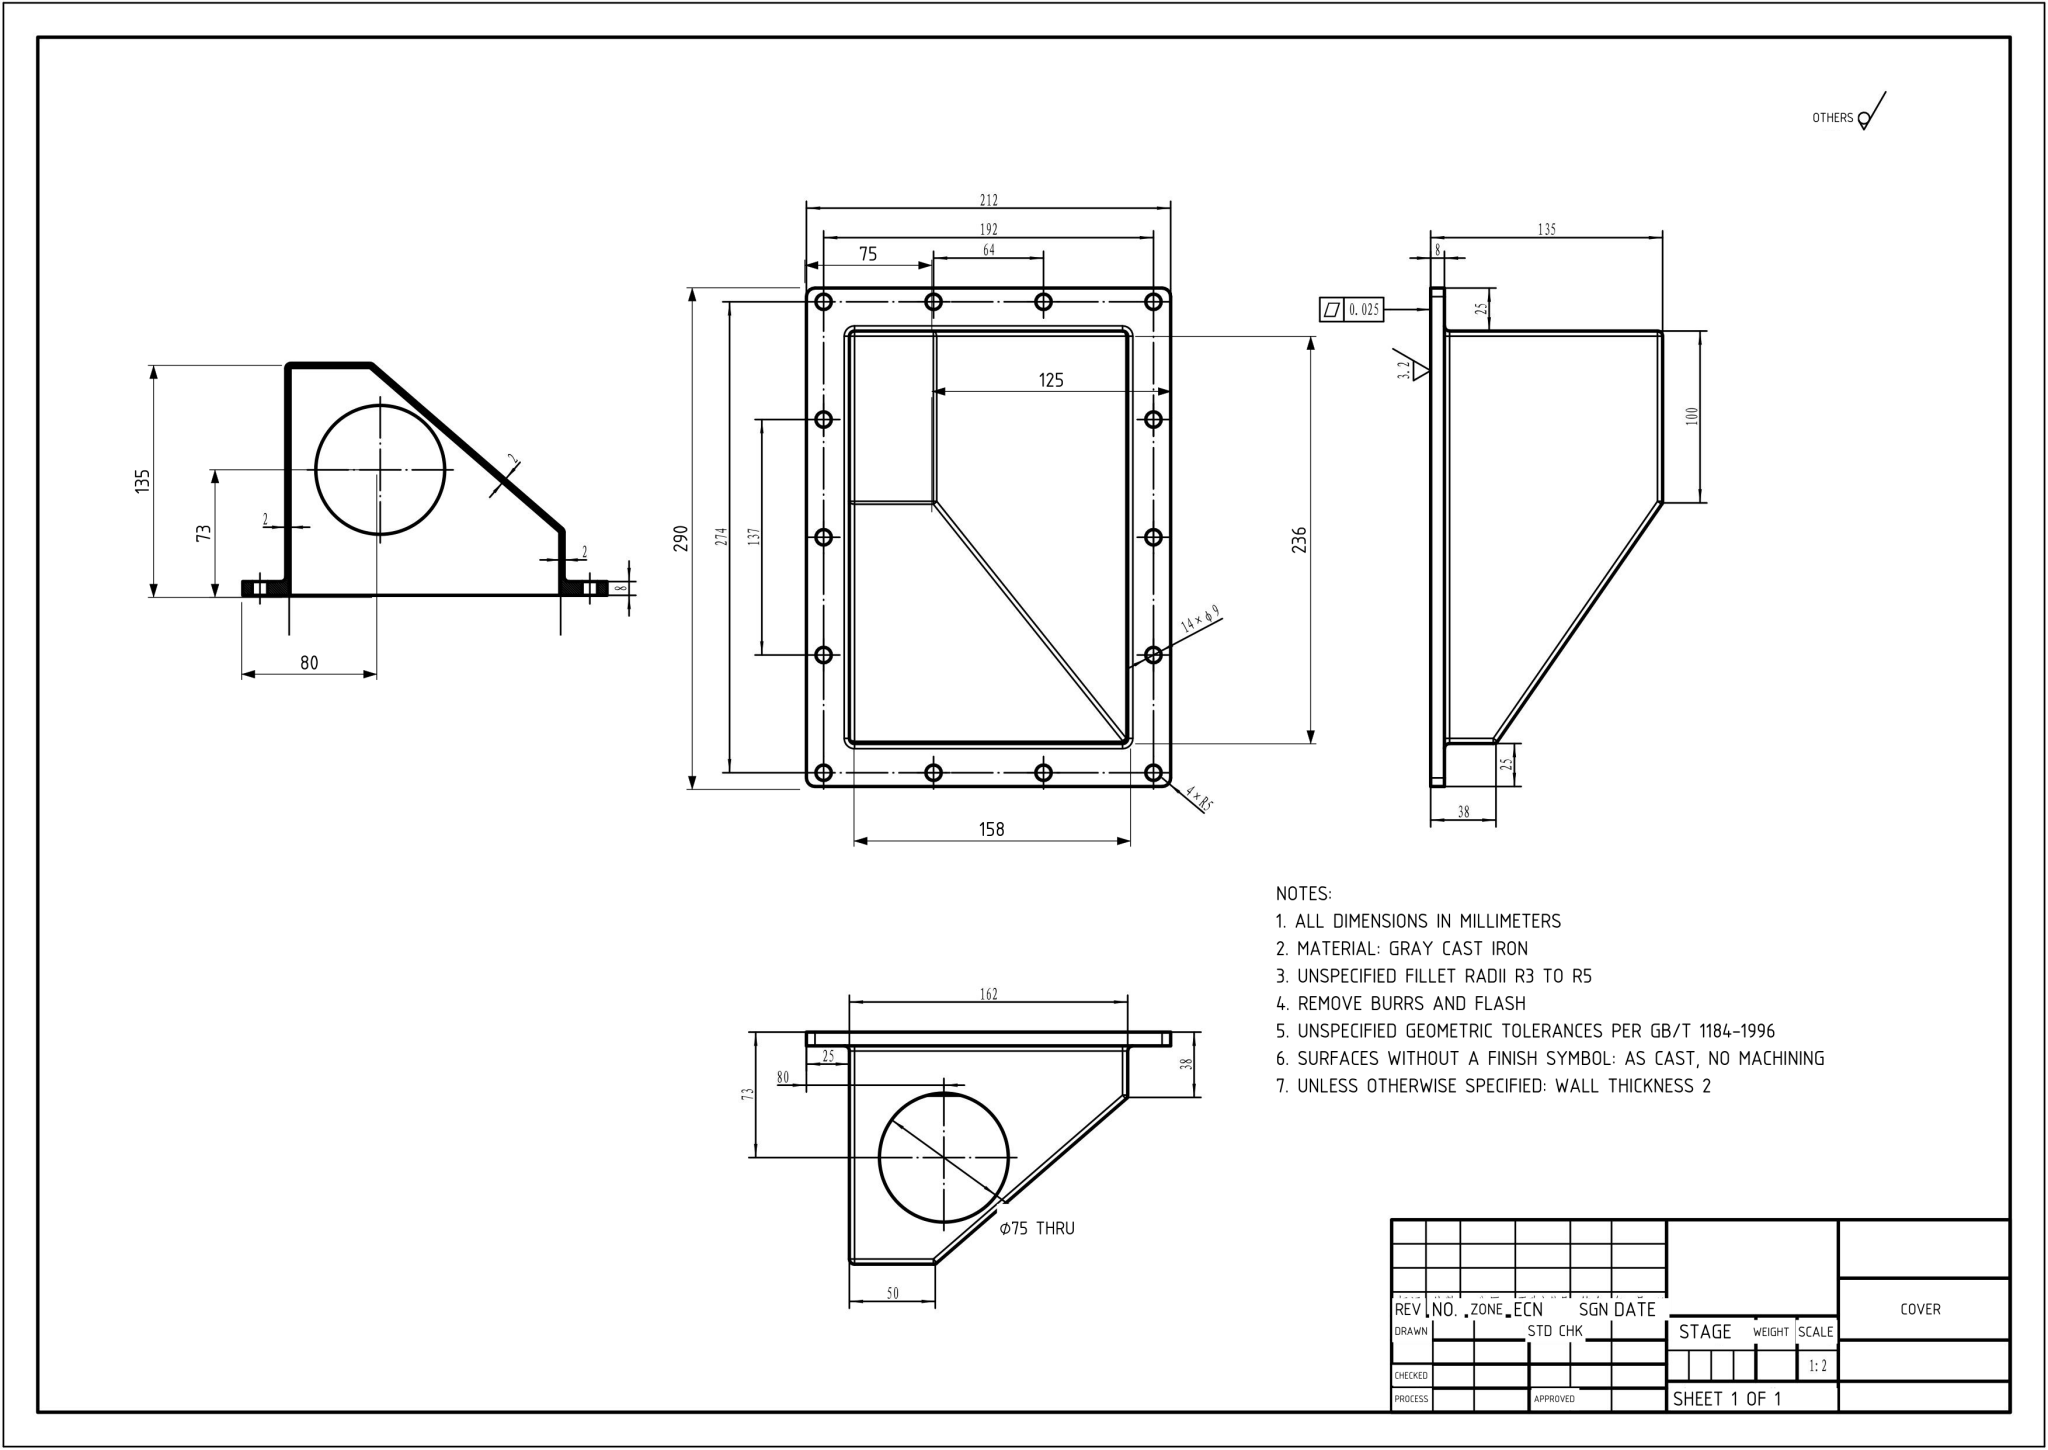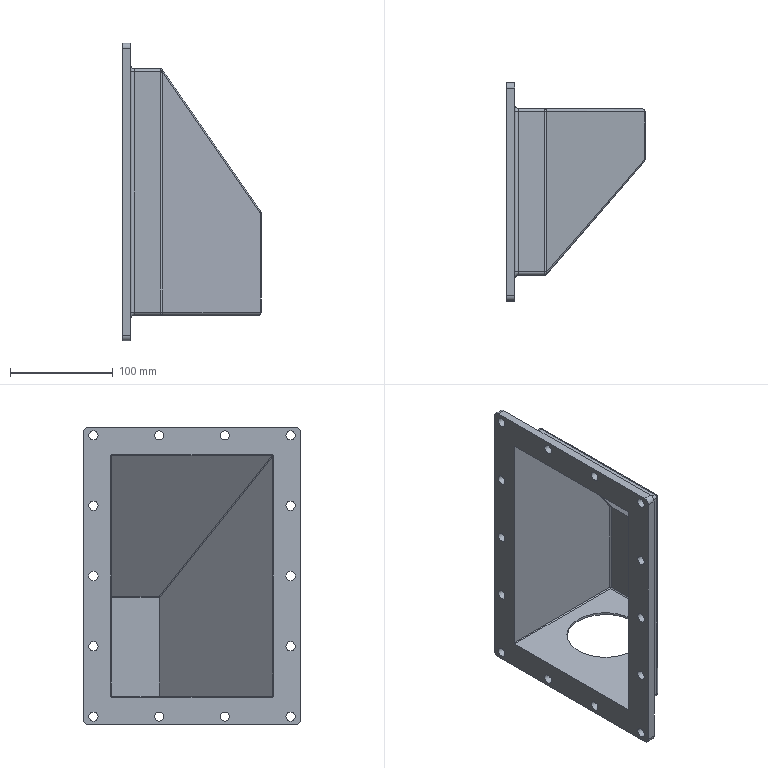Part | NX | mm | 1 solid | 91 faces | box 135 x 212 x 290 mm | volume 371782 mm3 | cylinder 51 | plane 20 | sphere 16 | torus 4 | commonest cylinder face diameters 6 x18 2 x14 9 x14 10 x4 75 x1